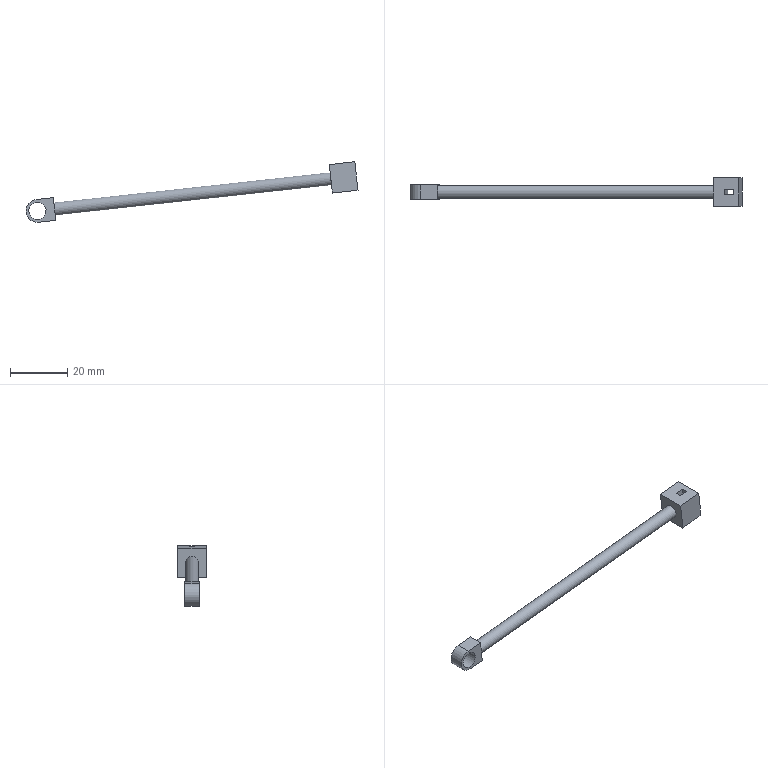Component | NX | LINK_3 | 1 solid | 18 faces | volume 2607 mm3 | plane 15 | cylinder 3 | commonest cylinder face diameters 4.5 x1 8 x1 6 x1